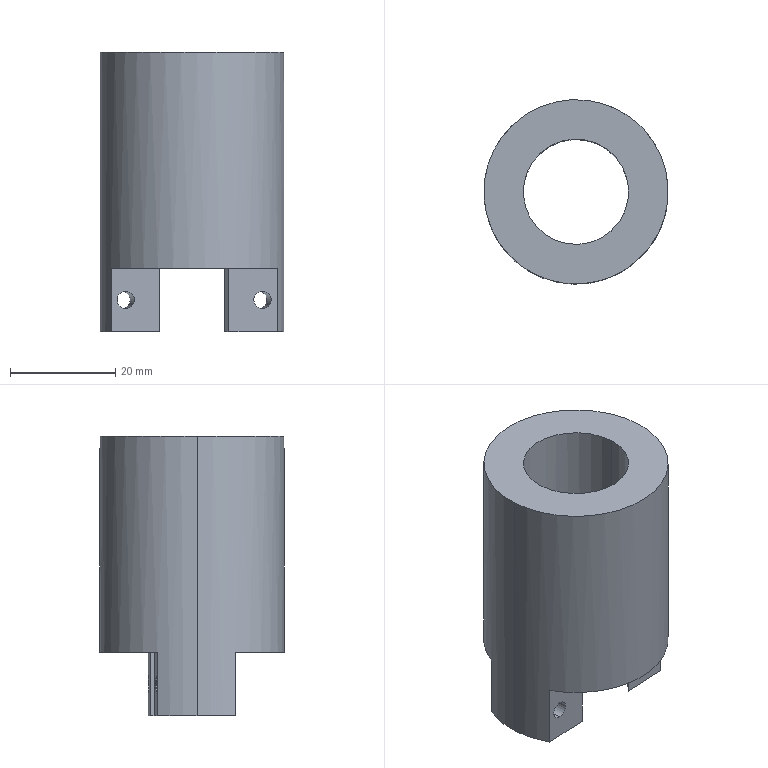Component | SolidWorks | BearingPressPartL-1 | 1 solid | 17 faces | box 35 x 35 x 53 mm | volume 29185 mm3 | plane 9 | cylinder 8 | commonest cylinder face diameters 3.3 x4 20 x2 35 x2
build123d program:
from build123d import *

# Parameters (mm, degrees)
SKETCH1_R           = 17.5
SKETCH1_R_2         = 10
BOSS_EXTRUDE1_DEPTH = 53
SKETCH2_W           = 66.079
SKETCH2_H           = 14.313
SKETCH2_H_2         = 17.096
CUT_EXTRUDE1_DEPTH  = 12
M4_TAPPED_HOLE1_D   = 3.3


with BuildPart() as part:
    # Sketch1 → Boss-Extrude1 (new body)
    with BuildSketch(Plane.XY):
        Circle(SKETCH1_R)
        Circle(SKETCH1_R_2, mode=Mode.SUBTRACT)
    extrude(amount=BOSS_EXTRUDE1_DEPTH)

    # Sketch2 → Cut-Extrude1 (cut)
    with BuildSketch(Plane(origin=(0, 0, 0), x_dir=(-1, 0, 0), z_dir=(0, 0, -1))):
        with Locations((0.159, 14.657)):
            Rectangle(SKETCH2_W, SKETCH2_H)
        with Locations((0.159, -16.048)):
            Rectangle(SKETCH2_W, SKETCH2_H_2)
    extrude(amount=-CUT_EXTRUDE1_DEPTH, mode=Mode.SUBTRACT)

    # M4 Tapped Hole1 (through all)
    with Locations(Plane(origin=(0, 7.5, 0), x_dir=(-1, 0, 0), z_dir=(0, 1, 0))):
        with Locations((-13, 6), (13, 6)):
            Hole(M4_TAPPED_HOLE1_D / 2)


solid = part.part

# Placed as in the assembly
solid = solid.moved(Location((447.676, 127.964, -295.818), (0, 0, -176.863)))
STEP:
#1=CARTESIAN_POINT('',(18.152,4.771,-11.475));
#2=VERTEX_POINT('',#1);
#3=CARTESIAN_POINT('',(18.152,4.771,-11.345));
#4=VERTEX_POINT('',#3);
#5=CARTESIAN_POINT('',(18.152,4.771,-11.41));
#6=DIRECTION('',(-0.05472,0.9985,0.));
#7=DIRECTION('',(0.,0.,1.));
#8=AXIS2_PLACEMENT_3D('',#5,#6,#7);
#9=CIRCLE('',#8,0.06496);
#10=EDGE_CURVE('',#2,#4,#9,.T.);
#11=ORIENTED_EDGE('',*,*,#10,.F.);
#12=CARTESIAN_POINT('',(18.12,5.361,-11.475));
#13=VERTEX_POINT('',#12);
#14=CARTESIAN_POINT('',(18.12,5.361,-11.475));
#15=DIRECTION('',(-0.05472,0.9985,0.));
#16=VECTOR('',#15,39.37);
#17=LINE('',#14,#16);
#18=EDGE_CURVE('',#2,#13,#17,.T.);
#19=ORIENTED_EDGE('',*,*,#18,.T.);
#20=CARTESIAN_POINT('',(18.12,5.361,-11.345));
#21=VERTEX_POINT('',#20);
#22=CARTESIAN_POINT('',(18.12,5.361,-11.41));
#23=DIRECTION('',(-0.05472,0.9985,0.));
#24=DIRECTION('',(0.,0.,1.));
#25=AXIS2_PLACEMENT_3D('',#22,#23,#24);
#26=CIRCLE('',#25,0.06496);
#27=EDGE_CURVE('',#13,#21,#26,.T.);
#28=ORIENTED_EDGE('',*,*,#27,.T.);
#29=CARTESIAN_POINT('',(18.12,5.361,-11.345));
#30=DIRECTION('',(-0.05472,0.9985,0.));
#31=VECTOR('',#30,39.37);
#32=LINE('',#29,#31);
#33=EDGE_CURVE('',#4,#21,#32,.T.);
#34=ORIENTED_EDGE('',*,*,#33,.F.);
#35=EDGE_LOOP('',(#11,#19,#28,#34));
#36=FACE_OUTER_BOUND('',#35,.T.);
#37=CARTESIAN_POINT('',(18.12,5.361,-11.41));
#38=DIRECTION('',(-0.05472,0.9985,0.));
#39=DIRECTION('',(0.,0.,1.));
#40=AXIS2_PLACEMENT_3D('',#37,#38,#39);
#41=CYLINDRICAL_SURFACE('',#40,0.06496);
#42=ADVANCED_FACE('',(#36),#41,.F.);
#43=CARTESIAN_POINT('',(17.13,4.715,-11.475));
#44=VERTEX_POINT('',#43);
#45=CARTESIAN_POINT('',(17.13,4.715,-11.345));
#46=VERTEX_POINT('',#45);
#47=CARTESIAN_POINT('',(17.13,4.715,-11.41));
#48=DIRECTION('',(-0.05472,0.9985,0.));
#49=DIRECTION('',(0.,0.,1.));
#50=AXIS2_PLACEMENT_3D('',#47,#48,#49);
#51=CIRCLE('',#50,0.06496);
#52=EDGE_CURVE('',#44,#46,#51,.T.);
#53=ORIENTED_EDGE('',*,*,#52,.F.);
#54=CARTESIAN_POINT('',(17.098,5.305,-11.475));
#55=VERTEX_POINT('',#54);
#56=CARTESIAN_POINT('',(17.098,5.305,-11.475));
#57=DIRECTION('',(-0.05472,0.9985,0.));
#58=VECTOR('',#57,39.37);
#59=LINE('',#56,#58);
#60=EDGE_CURVE('',#44,#55,#59,.T.);
#61=ORIENTED_EDGE('',*,*,#60,.T.);
#62=CARTESIAN_POINT('',(17.098,5.305,-11.345));
#63=VERTEX_POINT('',#62);
#64=CARTESIAN_POINT('',(17.098,5.305,-11.41));
#65=DIRECTION('',(-0.05472,0.9985,0.));
#66=DIRECTION('',(0.,0.,1.));
#67=AXIS2_PLACEMENT_3D('',#64,#65,#66);
#68=CIRCLE('',#67,0.06496);
#69=EDGE_CURVE('',#55,#63,#68,.T.);
#70=ORIENTED_EDGE('',*,*,#69,.T.);
#71=CARTESIAN_POINT('',(17.098,5.305,-11.345));
#72=DIRECTION('',(-0.05472,0.9985,0.));
#73=VECTOR('',#72,39.37);
#74=LINE('',#71,#73);
#75=EDGE_CURVE('',#46,#63,#74,.T.);
#76=ORIENTED_EDGE('',*,*,#75,.F.);
#77=EDGE_LOOP('',(#53,#61,#70,#76));
#78=FACE_OUTER_BOUND('',#77,.T.);
#79=CARTESIAN_POINT('',(17.098,5.305,-11.41));
#80=DIRECTION('',(-0.05472,0.9985,0.));
#81=DIRECTION('',(0.,0.,1.));
#82=AXIS2_PLACEMENT_3D('',#79,#80,#81);
#83=CYLINDRICAL_SURFACE('',#82,0.06496);
#84=ADVANCED_FACE('',(#78),#83,.F.);
#85=CARTESIAN_POINT('',(17.232,5.016,-9.56));
#86=VERTEX_POINT('',#85);
#87=CARTESIAN_POINT('',(18.018,5.059,-9.56));
#88=VERTEX_POINT('',#87);
#89=CARTESIAN_POINT('',(17.625,5.038,-9.56));
#90=DIRECTION('',(0.,0.,1.));
#91=DIRECTION('',(0.9985,0.05472,0.));
#92=AXIS2_PLACEMENT_3D('',#89,#90,#91);
#93=CIRCLE('',#92,0.3937);
#94=EDGE_CURVE('',#86,#88,#93,.T.);
#95=ORIENTED_EDGE('',*,*,#94,.T.);
#96=CARTESIAN_POINT('',(18.018,5.059,-11.646));
#97=VERTEX_POINT('',#96);
#98=CARTESIAN_POINT('',(18.018,5.059,-9.56));
#99=DIRECTION('',(0.,0.,-1.));
#100=VECTOR('',#99,39.37);
#101=LINE('',#98,#100);
#102=EDGE_CURVE('',#88,#97,#101,.T.);
#103=ORIENTED_EDGE('',*,*,#102,.T.);
#104=CARTESIAN_POINT('',(17.901,4.757,-11.646));
#105=VERTEX_POINT('',#104);
#106=CARTESIAN_POINT('',(17.625,5.038,-11.646));
#107=DIRECTION('',(0.,0.,1.));
#108=DIRECTION('',(0.9985,0.05472,0.));
#109=AXIS2_PLACEMENT_3D('',#106,#107,#108);
#110=CIRCLE('',#109,0.3937);
#111=EDGE_CURVE('',#105,#97,#110,.T.);
#112=ORIENTED_EDGE('',*,*,#111,.F.);
#113=CARTESIAN_POINT('',(17.901,4.757,-11.174));
#114=VERTEX_POINT('',#113);
#115=CARTESIAN_POINT('',(17.901,4.757,-9.56));
#116=DIRECTION('',(0.,0.,-1.));
#117=VECTOR('',#116,39.37);
#118=LINE('',#115,#117);
#119=EDGE_CURVE('',#114,#105,#118,.T.);
#120=ORIENTED_EDGE('',*,*,#119,.F.);
#121=CARTESIAN_POINT('',(17.381,4.729,-11.174));
#122=VERTEX_POINT('',#121);
#123=CARTESIAN_POINT('',(17.625,5.038,-11.174));
#124=DIRECTION('',(0.,0.,-1.));
#125=DIRECTION('',(-0.9985,-0.05472,0.));
#126=AXIS2_PLACEMENT_3D('',#123,#124,#125);
#127=CIRCLE('',#126,0.3937);
#128=EDGE_CURVE('',#114,#122,#127,.T.);
#129=ORIENTED_EDGE('',*,*,#128,.T.);
#130=CARTESIAN_POINT('',(17.381,4.729,-11.646));
#131=VERTEX_POINT('',#130);
#132=CARTESIAN_POINT('',(17.381,4.729,-9.56));
#133=DIRECTION('',(0.,0.,1.));
#134=VECTOR('',#133,39.37);
#135=LINE('',#132,#134);
#136=EDGE_CURVE('',#131,#122,#135,.T.);
#137=ORIENTED_EDGE('',*,*,#136,.F.);
#138=CARTESIAN_POINT('',(17.232,5.016,-11.646));
#139=VERTEX_POINT('',#138);
#140=CARTESIAN_POINT('',(17.625,5.038,-11.646));
#141=DIRECTION('',(0.,0.,1.));
#142=DIRECTION('',(0.9985,0.05472,0.));
#143=AXIS2_PLACEMENT_3D('',#140,#141,#142);
#144=CIRCLE('',#143,0.3937);
#145=EDGE_CURVE('',#139,#131,#144,.T.);
#146=ORIENTED_EDGE('',*,*,#145,.F.);
#147=CARTESIAN_POINT('',(17.232,5.016,-9.56));
#148=DIRECTION('',(0.,0.,-1.));
#149=VECTOR('',#148,39.37);
#150=LINE('',#147,#149);
#151=EDGE_CURVE('',#86,#139,#150,.T.);
#152=ORIENTED_EDGE('',*,*,#151,.F.);
#153=EDGE_LOOP('',(#95,#103,#112,#120,#129,#137,#146,#152));
#154=FACE_OUTER_BOUND('',#153,.T.);
#155=CARTESIAN_POINT('',(17.625,5.038,-9.56));
#156=DIRECTION('',(0.,0.,-1.));
#157=DIRECTION('',(-0.9985,-0.05472,0.));
#158=AXIS2_PLACEMENT_3D('',#155,#156,#157);
#159=CYLINDRICAL_SURFACE('',#158,0.3937);
#160=ADVANCED_FACE('',(#154),#159,.F.);
#161=CARTESIAN_POINT('',(18.313,5.076,-9.56));
#162=VERTEX_POINT('',#161);
#163=CARTESIAN_POINT('',(16.937,5.,-9.56));
#164=VERTEX_POINT('',#163);
#165=CARTESIAN_POINT('',(17.625,5.038,-9.56));
#166=DIRECTION('',(0.,0.,1.));
#167=DIRECTION('',(0.9985,0.05472,0.));
#168=AXIS2_PLACEMENT_3D('',#165,#166,#167);
#169=CIRCLE('',#168,0.689);
#170=EDGE_CURVE('',#162,#164,#169,.T.);
#171=ORIENTED_EDGE('',*,*,#170,.F.);
#172=CARTESIAN_POINT('',(18.313,5.076,-11.646));
#173=VERTEX_POINT('',#172);
#174=CARTESIAN_POINT('',(18.313,5.076,-9.56));
#175=DIRECTION('',(0.,0.,-1.));
#176=VECTOR('',#175,39.37);
#177=LINE('',#174,#176);
#178=EDGE_CURVE('',#162,#173,#177,.T.);
#179=ORIENTED_EDGE('',*,*,#178,.T.);
#180=CARTESIAN_POINT('',(18.23,5.367,-11.646));
#181=VERTEX_POINT('',#180);
#182=CARTESIAN_POINT('',(17.625,5.038,-11.646));
#183=DIRECTION('',(0.,0.,1.));
#184=DIRECTION('',(0.9985,0.05472,0.));
#185=AXIS2_PLACEMENT_3D('',#182,#183,#184);
#186=CIRCLE('',#185,0.689);
#187=EDGE_CURVE('',#173,#181,#186,.T.);
#188=ORIENTED_EDGE('',*,*,#187,.T.);
#189=CARTESIAN_POINT('',(18.23,5.367,-11.174));
#190=VERTEX_POINT('',#189);
#191=CARTESIAN_POINT('',(18.23,5.367,-9.56));
#192=DIRECTION('',(0.,0.,1.));
#193=VECTOR('',#192,39.37);
#194=LINE('',#191,#193);
#195=EDGE_CURVE('',#181,#190,#194,.T.);
#196=ORIENTED_EDGE('',*,*,#195,.T.);
#197=CARTESIAN_POINT('',(16.987,5.299,-11.174));
#198=VERTEX_POINT('',#197);
#199=CARTESIAN_POINT('',(17.625,5.038,-11.174));
#200=DIRECTION('',(0.,0.,-1.));
#201=DIRECTION('',(-0.9985,-0.05472,0.));
#202=AXIS2_PLACEMENT_3D('',#199,#200,#201);
#203=CIRCLE('',#202,0.689);
#204=EDGE_CURVE('',#198,#190,#203,.T.);
#205=ORIENTED_EDGE('',*,*,#204,.F.);
#206=CARTESIAN_POINT('',(16.987,5.299,-11.646));
#207=VERTEX_POINT('',#206);
#208=CARTESIAN_POINT('',(16.987,5.299,-9.56));
#209=DIRECTION('',(0.,0.,-1.));
#210=VECTOR('',#209,39.37);
#211=LINE('',#208,#210);
#212=EDGE_CURVE('',#198,#207,#211,.T.);
#213=ORIENTED_EDGE('',*,*,#212,.T.);
#214=CARTESIAN_POINT('',(16.937,5.,-11.646));
#215=VERTEX_POINT('',#214);
#216=CARTESIAN_POINT('',(17.625,5.038,-11.646));
#217=DIRECTION('',(0.,0.,1.));
#218=DIRECTION('',(0.9985,0.05472,0.));
#219=AXIS2_PLACEMENT_3D('',#216,#217,#218);
#220=CIRCLE('',#219,0.689);
#221=EDGE_CURVE('',#207,#215,#220,.T.);
#222=ORIENTED_EDGE('',*,*,#221,.T.);
#223=CARTESIAN_POINT('',(16.937,5.,-9.56));
#224=DIRECTION('',(0.,0.,-1.));
#225=VECTOR('',#224,39.37);
#226=LINE('',#223,#225);
#227=EDGE_CURVE('',#164,#215,#226,.T.);
#228=ORIENTED_EDGE('',*,*,#227,.F.);
#229=EDGE_LOOP('',(#171,#179,#188,#196,#205,#213,#222,#228));
#230=FACE_OUTER_BOUND('',#229,.T.);
#231=CARTESIAN_POINT('',(17.625,5.038,-9.56));
#232=DIRECTION('',(0.,0.,-1.));
#233=DIRECTION('',(-0.9985,-0.05472,0.));
#234=AXIS2_PLACEMENT_3D('',#231,#232,#233);
#235=CYLINDRICAL_SURFACE('',#234,0.689);
#236=ADVANCED_FACE('',(#230),#235,.T.);
#237=ORIENTED_EDGE('',*,*,#221,.F.);
#238=CARTESIAN_POINT('',(17.349,5.319,-11.646));
#239=VERTEX_POINT('',#238);
#240=CARTESIAN_POINT('',(18.901,5.404,-11.646));
#241=DIRECTION('',(-0.9985,-0.05472,0.));
#242=VECTOR('',#241,39.37);
#243=LINE('',#240,#242);
#244=EDGE_CURVE('',#239,#207,#243,.T.);
#245=ORIENTED_EDGE('',*,*,#244,.F.);
#246=CARTESIAN_POINT('',(17.625,5.038,-11.646));
#247=DIRECTION('',(0.,0.,1.));
#248=DIRECTION('',(0.9985,0.05472,0.));
#249=AXIS2_PLACEMENT_3D('',#246,#247,#248);
#250=CIRCLE('',#249,0.3937);
#251=EDGE_CURVE('',#239,#139,#250,.T.);
#252=ORIENTED_EDGE('',*,*,#251,.T.);
#253=ORIENTED_EDGE('',*,*,#145,.T.);
#254=CARTESIAN_POINT('',(17.02,4.709,-11.646));
#255=VERTEX_POINT('',#254);
#256=CARTESIAN_POINT('',(18.934,4.814,-11.646));
#257=DIRECTION('',(0.9985,0.05472,0.));
#258=VECTOR('',#257,39.37);
#259=LINE('',#256,#258);
#260=EDGE_CURVE('',#255,#131,#259,.T.);
#261=ORIENTED_EDGE('',*,*,#260,.F.);
#262=CARTESIAN_POINT('',(17.625,5.038,-11.646));
#263=DIRECTION('',(0.,0.,1.));
#264=DIRECTION('',(0.9985,0.05472,0.));
#265=AXIS2_PLACEMENT_3D('',#262,#263,#264);
#266=CIRCLE('',#265,0.689);
#267=EDGE_CURVE('',#215,#255,#266,.T.);
#268=ORIENTED_EDGE('',*,*,#267,.F.);
#269=EDGE_LOOP('',(#237,#245,#252,#253,#261,#268));
#270=FACE_OUTER_BOUND('',#269,.T.);
#271=CARTESIAN_POINT('',(17.625,5.038,-11.646));
#272=DIRECTION('',(0.,0.,1.));
#273=DIRECTION('',(0.9985,0.05472,0.));
#274=AXIS2_PLACEMENT_3D('',#271,#272,#273);
#275=PLANE('',#274);
#276=ADVANCED_FACE('',(#270),#275,.F.);
#277=CARTESIAN_POINT('',(17.625,5.038,-9.56));
#278=DIRECTION('',(0.,0.,1.));
#279=DIRECTION('',(0.9985,0.05472,0.));
#280=AXIS2_PLACEMENT_3D('',#277,#278,#279);
#281=CIRCLE('',#280,0.689);
#282=EDGE_CURVE('',#164,#162,#281,.T.);
#283=ORIENTED_EDGE('',*,*,#282,.T.);
#284=ORIENTED_EDGE('',*,*,#170,.T.);
#285=EDGE_LOOP('',(#283,#284));
#286=FACE_OUTER_BOUND('',#285,.T.);
#287=ORIENTED_EDGE('',*,*,#94,.F.);
#288=CARTESIAN_POINT('',(17.625,5.038,-9.56));
#289=DIRECTION('',(0.,0.,1.));
#290=DIRECTION('',(0.9985,0.05472,0.));
#291=AXIS2_PLACEMENT_3D('',#288,#289,#290);
#292=CIRCLE('',#291,0.3937);
#293=EDGE_CURVE('',#88,#86,#292,.T.);
#294=ORIENTED_EDGE('',*,*,#293,.F.);
#295=EDGE_LOOP('',(#287,#294));
#296=FACE_BOUND('',#295,.T.);
#297=CARTESIAN_POINT('',(17.625,5.038,-9.56));
#298=DIRECTION('',(0.,0.,1.));
#299=DIRECTION('',(0.9985,0.05472,0.));
#300=AXIS2_PLACEMENT_3D('',#297,#298,#299);
#301=PLANE('',#300);
#302=ADVANCED_FACE('',(#286,#296),#301,.T.);
#303=ORIENTED_EDGE('',*,*,#111,.T.);
#304=CARTESIAN_POINT('',(17.869,5.347,-11.646));
#305=VERTEX_POINT('',#304);
#306=CARTESIAN_POINT('',(17.625,5.038,-11.646));
#307=DIRECTION('',(0.,0.,1.));
#308=DIRECTION('',(0.9985,0.05472,0.));
#309=AXIS2_PLACEMENT_3D('',#306,#307,#308);
#310=CIRCLE('',#309,0.3937);
#311=EDGE_CURVE('',#97,#305,#310,.T.);
#312=ORIENTED_EDGE('',*,*,#311,.T.);
#313=CARTESIAN_POINT('',(18.901,5.404,-11.646));
#314=DIRECTION('',(-0.9985,-0.05472,0.));
#315=VECTOR('',#314,39.37);
#316=LINE('',#313,#315);
#317=EDGE_CURVE('',#181,#305,#316,.T.);
#318=ORIENTED_EDGE('',*,*,#317,.F.);
#319=ORIENTED_EDGE('',*,*,#187,.F.);
#320=CARTESIAN_POINT('',(18.263,4.777,-11.646));
#321=VERTEX_POINT('',#320);
#322=CARTESIAN_POINT('',(17.625,5.038,-11.646));
#323=DIRECTION('',(0.,0.,1.));
#324=DIRECTION('',(0.9985,0.05472,0.));
#325=AXIS2_PLACEMENT_3D('',#322,#323,#324);
#326=CIRCLE('',#325,0.689);
#327=EDGE_CURVE('',#321,#173,#326,.T.);
#328=ORIENTED_EDGE('',*,*,#327,.F.);
#329=CARTESIAN_POINT('',(18.934,4.814,-11.646));
#330=DIRECTION('',(0.9985,0.05472,0.));
#331=VECTOR('',#330,39.37);
#332=LINE('',#329,#331);
#333=EDGE_CURVE('',#105,#321,#332,.T.);
#334=ORIENTED_EDGE('',*,*,#333,.F.);
#335=EDGE_LOOP('',(#303,#312,#318,#319,#328,#334));
#336=FACE_OUTER_BOUND('',#335,.T.);
#337=CARTESIAN_POINT('',(17.625,5.038,-11.646));
#338=DIRECTION('',(0.,0.,1.));
#339=DIRECTION('',(0.9985,0.05472,0.));
#340=AXIS2_PLACEMENT_3D('',#337,#338,#339);
#341=PLANE('',#340);
#342=ADVANCED_FACE('',(#336),#341,.F.);
#343=ORIENTED_EDGE('',*,*,#178,.F.);
#344=ORIENTED_EDGE('',*,*,#282,.F.);
#345=ORIENTED_EDGE('',*,*,#227,.T.);
#346=ORIENTED_EDGE('',*,*,#267,.T.);
#347=CARTESIAN_POINT('',(17.02,4.709,-11.174));
#348=VERTEX_POINT('',#347);
#349=CARTESIAN_POINT('',(17.02,4.709,-9.56));
#350=DIRECTION('',(0.,0.,1.));
#351=VECTOR('',#350,39.37);
#352=LINE('',#349,#351);
#353=EDGE_CURVE('',#255,#348,#352,.T.);
#354=ORIENTED_EDGE('',*,*,#353,.T.);
#355=CARTESIAN_POINT('',(18.263,4.777,-11.174));
#356=VERTEX_POINT('',#355);
#357=CARTESIAN_POINT('',(17.625,5.038,-11.174));
#358=DIRECTION('',(0.,0.,-1.));
#359=DIRECTION('',(-0.9985,-0.05472,0.));
#360=AXIS2_PLACEMENT_3D('',#357,#358,#359);
#361=CIRCLE('',#360,0.689);
#362=EDGE_CURVE('',#356,#348,#361,.T.);
#363=ORIENTED_EDGE('',*,*,#362,.F.);
#364=CARTESIAN_POINT('',(18.263,4.777,-9.56));
#365=DIRECTION('',(0.,0.,-1.));
#366=VECTOR('',#365,39.37);
#367=LINE('',#364,#366);
#368=EDGE_CURVE('',#356,#321,#367,.T.);
#369=ORIENTED_EDGE('',*,*,#368,.T.);
#370=ORIENTED_EDGE('',*,*,#327,.T.);
#371=EDGE_LOOP('',(#343,#344,#345,#346,#354,#363,#369,#370));
#372=FACE_OUTER_BOUND('',#371,.T.);
#373=CARTESIAN_POINT('',(17.625,5.038,-9.56));
#374=DIRECTION('',(0.,0.,-1.));
#375=DIRECTION('',(-0.9985,-0.05472,0.));
#376=AXIS2_PLACEMENT_3D('',#373,#374,#375);
#377=CYLINDRICAL_SURFACE('',#376,0.689);
#378=ADVANCED_FACE('',(#372),#377,.T.);
#379=ORIENTED_EDGE('',*,*,#102,.F.);
#380=ORIENTED_EDGE('',*,*,#293,.T.);
#381=ORIENTED_EDGE('',*,*,#151,.T.);
#382=ORIENTED_EDGE('',*,*,#251,.F.);
#383=CARTESIAN_POINT('',(17.349,5.319,-11.174));
#384=VERTEX_POINT('',#383);
#385=CARTESIAN_POINT('',(17.349,5.319,-9.56));
#386=DIRECTION('',(0.,0.,-1.));
#387=VECTOR('',#386,39.37);
#388=LINE('',#385,#387);
#389=EDGE_CURVE('',#384,#239,#388,.T.);
#390=ORIENTED_EDGE('',*,*,#389,.F.);
#391=CARTESIAN_POINT('',(17.869,5.347,-11.174));
#392=VERTEX_POINT('',#391);
#393=CARTESIAN_POINT('',(17.625,5.038,-11.174));
#394=DIRECTION('',(0.,0.,-1.));
#395=DIRECTION('',(-0.9985,-0.05472,0.));
#396=AXIS2_PLACEMENT_3D('',#393,#394,#395);
#397=CIRCLE('',#396,0.3937);
#398=EDGE_CURVE('',#384,#392,#397,.T.);
#399=ORIENTED_EDGE('',*,*,#398,.T.);
#400=CARTESIAN_POINT('',(17.869,5.347,-9.56));
#401=DIRECTION('',(0.,0.,1.));
#402=VECTOR('',#401,39.37);
#403=LINE('',#400,#402);
#404=EDGE_CURVE('',#305,#392,#403,.T.);
#405=ORIENTED_EDGE('',*,*,#404,.F.);
#406=ORIENTED_EDGE('',*,*,#311,.F.);
#407=EDGE_LOOP('',(#379,#380,#381,#382,#390,#399,#405,#406));
#408=FACE_OUTER_BOUND('',#407,.T.);
#409=CARTESIAN_POINT('',(17.625,5.038,-9.56));
#410=DIRECTION('',(0.,0.,-1.));
#411=DIRECTION('',(-0.9985,-0.05472,0.));
#412=AXIS2_PLACEMENT_3D('',#409,#410,#411);
#413=CYLINDRICAL_SURFACE('',#412,0.3937);
#414=ADVANCED_FACE('',(#408),#413,.F.);
#415=CARTESIAN_POINT('',(18.152,4.771,-11.41));
#416=DIRECTION('',(-0.05472,0.9985,0.));
#417=DIRECTION('',(0.,0.,1.));
#418=AXIS2_PLACEMENT_3D('',#415,#416,#417);
#419=CIRCLE('',#418,0.06496);
#420=EDGE_CURVE('',#4,#2,#419,.T.);
#421=ORIENTED_EDGE('',*,*,#420,.T.);
#422=ORIENTED_EDGE('',*,*,#10,.T.);
#423=EDGE_LOOP('',(#421,#422));
#424=FACE_BOUND('',#423,.T.);
#425=CARTESIAN_POINT('',(18.934,4.814,-11.174));
#426=DIRECTION('',(0.9985,0.05472,0.));
#427=VECTOR('',#426,39.37);
#428=LINE('',#425,#427);
#429=EDGE_CURVE('',#114,#356,#428,.T.);
#430=ORIENTED_EDGE('',*,*,#429,.F.);
#431=ORIENTED_EDGE('',*,*,#119,.T.);
#432=ORIENTED_EDGE('',*,*,#333,.T.);
#433=ORIENTED_EDGE('',*,*,#368,.F.);
#434=EDGE_LOOP('',(#430,#431,#432,#433));
#435=FACE_OUTER_BOUND('',#434,.T.);
#436=CARTESIAN_POINT('',(18.934,4.814,-11.174));
#437=DIRECTION('',(-0.05472,0.9985,0.));
#438=DIRECTION('',(0.,0.,1.));
#439=AXIS2_PLACEMENT_3D('',#436,#437,#438);
#440=PLANE('',#439);
#441=ADVANCED_FACE('',(#424,#435),#440,.F.);
#442=CARTESIAN_POINT('',(17.13,4.715,-11.41));
#443=DIRECTION('',(-0.05472,0.9985,0.));
#444=DIRECTION('',(0.,0.,1.));
#445=AXIS2_PLACEMENT_3D('',#442,#443,#444);
#446=CIRCLE('',#445,0.06496);
#447=EDGE_CURVE('',#46,#44,#446,.T.);
#448=ORIENTED_EDGE('',*,*,#447,.T.);
#449=ORIENTED_EDGE('',*,*,#52,.T.);
#450=EDGE_LOOP('',(#448,#449));
#451=FACE_BOUND('',#450,.T.);
#452=ORIENTED_EDGE('',*,*,#260,.T.);
#453=ORIENTED_EDGE('',*,*,#136,.T.);
#454=CARTESIAN_POINT('',(18.934,4.814,-11.174));
#455=DIRECTION('',(0.9985,0.05472,0.));
#456=VECTOR('',#455,39.37);
#457=LINE('',#454,#456);
#458=EDGE_CURVE('',#348,#122,#457,.T.);
#459=ORIENTED_EDGE('',*,*,#458,.F.);
#460=ORIENTED_EDGE('',*,*,#353,.F.);
#461=EDGE_LOOP('',(#452,#453,#459,#460));
#462=FACE_OUTER_BOUND('',#461,.T.);
#463=CARTESIAN_POINT('',(18.934,4.814,-11.174));
#464=DIRECTION('',(-0.05472,0.9985,0.));
#465=DIRECTION('',(0.,0.,1.));
#466=AXIS2_PLACEMENT_3D('',#463,#464,#465);
#467=PLANE('',#466);
#468=ADVANCED_FACE('',(#451,#462),#467,.F.);
#469=ORIENTED_EDGE('',*,*,#362,.T.);
#470=ORIENTED_EDGE('',*,*,#458,.T.);
#471=ORIENTED_EDGE('',*,*,#128,.F.);
#472=ORIENTED_EDGE('',*,*,#429,.T.);
#473=EDGE_LOOP('',(#469,#470,#471,#472));
#474=FACE_OUTER_BOUND('',#473,.T.);
#475=CARTESIAN_POINT('',(17.625,5.038,-11.174));
#476=DIRECTION('',(0.,0.,-1.));
#477=DIRECTION('',(-0.9985,-0.05472,0.));
#478=AXIS2_PLACEMENT_3D('',#475,#476,#477);
#479=PLANE('',#478);
#480=ADVANCED_FACE('',(#474),#479,.T.);
#481=CARTESIAN_POINT('',(17.098,5.305,-11.41));
#482=DIRECTION('',(-0.05472,0.9985,0.));
#483=DIRECTION('',(0.,0.,1.));
#484=AXIS2_PLACEMENT_3D('',#481,#482,#483);
#485=CIRCLE('',#484,0.06496);
#486=EDGE_CURVE('',#63,#55,#485,.T.);
#487=ORIENTED_EDGE('',*,*,#486,.F.);
#488=ORIENTED_EDGE('',*,*,#69,.F.);
#489=EDGE_LOOP('',(#487,#488));
#490=FACE_BOUND('',#489,.T.);
#491=CARTESIAN_POINT('',(18.901,5.404,-11.174));
#492=DIRECTION('',(-0.9985,-0.05472,0.));
#493=VECTOR('',#492,39.37);
#494=LINE('',#491,#493);
#495=EDGE_CURVE('',#384,#198,#494,.T.);
#496=ORIENTED_EDGE('',*,*,#495,.F.);
#497=ORIENTED_EDGE('',*,*,#389,.T.);
#498=ORIENTED_EDGE('',*,*,#244,.T.);
#499=ORIENTED_EDGE('',*,*,#212,.F.);
#500=EDGE_LOOP('',(#496,#497,#498,#499));
#501=FACE_OUTER_BOUND('',#500,.T.);
#502=CARTESIAN_POINT('',(18.901,5.404,-11.174));
#503=DIRECTION('',(0.05472,-0.9985,0.));
#504=DIRECTION('',(0.,0.,-1.));
#505=AXIS2_PLACEMENT_3D('',#502,#503,#504);
#506=PLANE('',#505);
#507=ADVANCED_FACE('',(#490,#501),#506,.F.);
#508=CARTESIAN_POINT('',(18.12,5.361,-11.41));
#509=DIRECTION('',(-0.05472,0.9985,0.));
#510=DIRECTION('',(0.,0.,1.));
#511=AXIS2_PLACEMENT_3D('',#508,#509,#510);
#512=CIRCLE('',#511,0.06496);
#513=EDGE_CURVE('',#21,#13,#512,.T.);
#514=ORIENTED_EDGE('',*,*,#513,.F.);
#515=ORIENTED_EDGE('',*,*,#27,.F.);
#516=EDGE_LOOP('',(#514,#515));
#517=FACE_BOUND('',#516,.T.);
#518=ORIENTED_EDGE('',*,*,#317,.T.);
#519=ORIENTED_EDGE('',*,*,#404,.T.);
#520=CARTESIAN_POINT('',(18.901,5.404,-11.174));
#521=DIRECTION('',(-0.9985,-0.05472,0.));
#522=VECTOR('',#521,39.37);
#523=LINE('',#520,#522);
#524=EDGE_CURVE('',#190,#392,#523,.T.);
#525=ORIENTED_EDGE('',*,*,#524,.F.);
#526=ORIENTED_EDGE('',*,*,#195,.F.);
#527=EDGE_LOOP('',(#518,#519,#525,#526));
#528=FACE_OUTER_BOUND('',#527,.T.);
#529=CARTESIAN_POINT('',(18.901,5.404,-11.174));
#530=DIRECTION('',(0.05472,-0.9985,0.));
#531=DIRECTION('',(0.,0.,-1.));
#532=AXIS2_PLACEMENT_3D('',#529,#530,#531);
#533=PLANE('',#532);
#534=ADVANCED_FACE('',(#517,#528),#533,.F.);
#535=ORIENTED_EDGE('',*,*,#204,.T.);
#536=ORIENTED_EDGE('',*,*,#524,.T.);
#537=ORIENTED_EDGE('',*,*,#398,.F.);
#538=ORIENTED_EDGE('',*,*,#495,.T.);
#539=EDGE_LOOP('',(#535,#536,#537,#538));
#540=FACE_OUTER_BOUND('',#539,.T.);
#541=CARTESIAN_POINT('',(17.625,5.038,-11.174));
#542=DIRECTION('',(0.,0.,-1.));
#543=DIRECTION('',(-0.9985,-0.05472,0.));
#544=AXIS2_PLACEMENT_3D('',#541,#542,#543);
#545=PLANE('',#544);
#546=ADVANCED_FACE('',(#540),#545,.T.);
#547=ORIENTED_EDGE('',*,*,#60,.F.);
#548=ORIENTED_EDGE('',*,*,#447,.F.);
#549=ORIENTED_EDGE('',*,*,#75,.T.);
#550=ORIENTED_EDGE('',*,*,#486,.T.);
#551=EDGE_LOOP('',(#547,#548,#549,#550));
#552=FACE_OUTER_BOUND('',#551,.T.);
#553=CARTESIAN_POINT('',(17.098,5.305,-11.41));
#554=DIRECTION('',(-0.05472,0.9985,0.));
#555=DIRECTION('',(0.,0.,1.));
#556=AXIS2_PLACEMENT_3D('',#553,#554,#555);
#557=CYLINDRICAL_SURFACE('',#556,0.06496);
#558=ADVANCED_FACE('',(#552),#557,.F.);
#559=ORIENTED_EDGE('',*,*,#18,.F.);
#560=ORIENTED_EDGE('',*,*,#420,.F.);
#561=ORIENTED_EDGE('',*,*,#33,.T.);
#562=ORIENTED_EDGE('',*,*,#513,.T.);
#563=EDGE_LOOP('',(#559,#560,#561,#562));
#564=FACE_OUTER_BOUND('',#563,.T.);
#565=CARTESIAN_POINT('',(18.12,5.361,-11.41));
#566=DIRECTION('',(-0.05472,0.9985,0.));
#567=DIRECTION('',(0.,0.,1.));
#568=AXIS2_PLACEMENT_3D('',#565,#566,#567);
#569=CYLINDRICAL_SURFACE('',#568,0.06496);
#570=ADVANCED_FACE('',(#564),#569,.F.);
#571=CLOSED_SHELL('',(#42,#84,#160,#236,#276,#302,#342,#378,#414,#441,#468,#480,#507,#534,#546,#558,#570));
#572=MANIFOLD_SOLID_BREP('',#571);
#573=CARTESIAN_POINT('',(0.,0.,0.));
#574=DIRECTION('',(0.,0.,1.));
#575=DIRECTION('',(1.,0.,0.));
#576=AXIS2_PLACEMENT_3D('',#573,#574,#575);
#577=(LENGTH_UNIT()NAMED_UNIT(*)SI_UNIT($,.METRE.));
#578=LENGTH_MEASURE_WITH_UNIT(LENGTH_MEASURE(0.0254),#577);
#579=DIMENSIONAL_EXPONENTS(1.,0.,0.,0.,0.,0.,0.);
#580=(CONVERSION_BASED_UNIT('',#578)LENGTH_UNIT()NAMED_UNIT(#579));
#581=UNCERTAINTY_MEASURE_WITH_UNIT(LENGTH_MEASURE(0.00001),#580,'','');
#582=(NAMED_UNIT(*)PLANE_ANGLE_UNIT()SI_UNIT($,.RADIAN.));
#583=(NAMED_UNIT(*)SI_UNIT($,.STERADIAN.)SOLID_ANGLE_UNIT());
#584=(GEOMETRIC_REPRESENTATION_CONTEXT(3)GLOBAL_UNCERTAINTY_ASSIGNED_CONTEXT((#581))GLOBAL_UNIT_ASSIGNED_CONTEXT((#580,#582,#583))REPRESENTATION_CONTEXT('',''));
#585=ADVANCED_BREP_SHAPE_REPRESENTATION('',(#572,#576),#584);
#586=COLOUR_RGB('',0.7922,0.8196,0.9333);
#587=FILL_AREA_STYLE_COLOUR('',#586);
#588=FILL_AREA_STYLE('',(#587));
#589=SURFACE_STYLE_FILL_AREA(#588);
#590=SURFACE_SIDE_STYLE('',(#589));
#591=SURFACE_STYLE_USAGE(.BOTH.,#590);
#592=PRESENTATION_STYLE_ASSIGNMENT((#591));
#593=STYLED_ITEM('',(#592),#572);
#594=PRESENTATION_LAYER_ASSIGNMENT('','',(#593));
#595=(LENGTH_UNIT()NAMED_UNIT(*)SI_UNIT($,.METRE.));
#596=LENGTH_MEASURE_WITH_UNIT(LENGTH_MEASURE(0.0254),#595);
#597=DIMENSIONAL_EXPONENTS(1.,0.,0.,0.,0.,0.,0.);
#598=(CONVERSION_BASED_UNIT('',#596)LENGTH_UNIT()NAMED_UNIT(#597));
#599=UNCERTAINTY_MEASURE_WITH_UNIT(LENGTH_MEASURE(0.00001),#598,'','');
#600=(NAMED_UNIT(*)PLANE_ANGLE_UNIT()SI_UNIT($,.RADIAN.));
#601=(NAMED_UNIT(*)SI_UNIT($,.STERADIAN.)SOLID_ANGLE_UNIT());
#602=(GEOMETRIC_REPRESENTATION_CONTEXT(3)GLOBAL_UNCERTAINTY_ASSIGNED_CONTEXT((#599))GLOBAL_UNIT_ASSIGNED_CONTEXT((#598,#600,#601))REPRESENTATION_CONTEXT('',''));
#603=MECHANICAL_DESIGN_GEOMETRIC_PRESENTATION_REPRESENTATION('',(#593),#602);